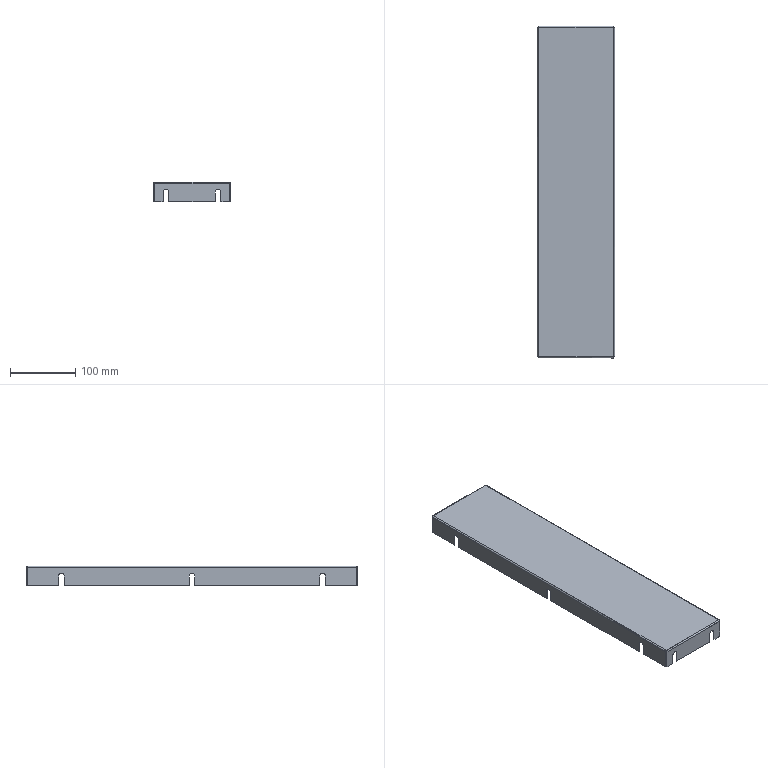Component | SolidWorks | SheetMetal120x510-1 | 1 solid | 88 faces | volume 111935 mm3 | plane 52 | cylinder 28 | spline 8 | commonest cylinder face diameters 8.5 x20 3.873 x4 1.473 x4